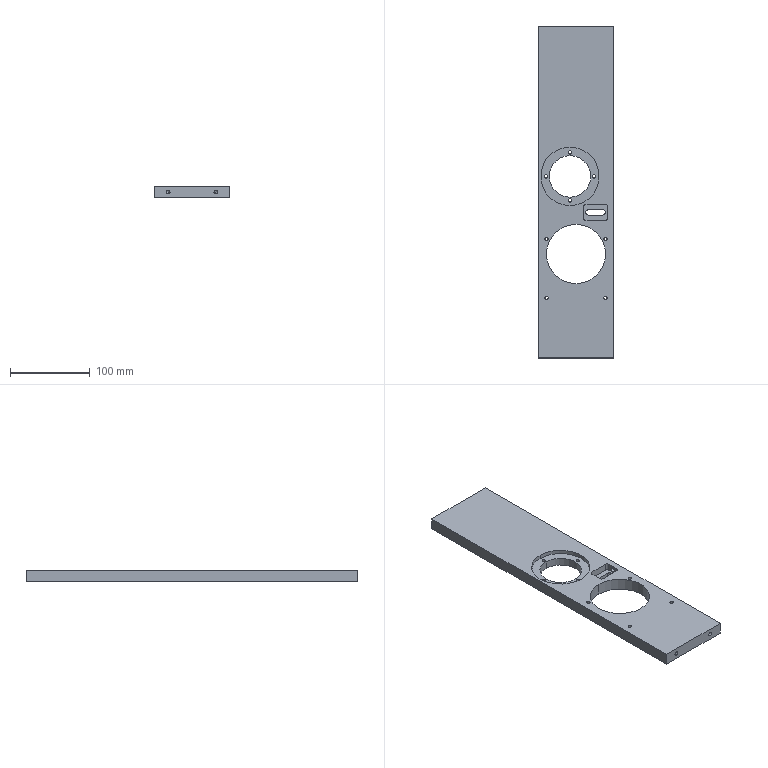Component | SolidWorks | 8TC-A15004-D0-02A-2 | 1 solid | 76 faces | box 95 x 415 x 15 mm | volume 474411 mm3 | cylinder 46 | cone 16 | plane 14 | commonest cylinder face diameters 5 x18 4.2 x16 6 x4 73 x2 74 x2 52 x2 6.5 x2 | material #45
build123d program:
from build123d import *

# Parameters (mm, degrees)
SKETCH1_W             = 95
SKETCH1_H             = 415
BOSS_EXTRUDE1_DEPTH   = 7.5
SKETCH3_R             = 26
CUT_EXTRUDE2_DEPTH    = 214.395
SKETCH4_R             = 37
CUT_EXTRUDE3_DEPTH    = 214.395
SKETCH5_R             = 36.5
CUT_EXTRUDE4_DEPTH    = 5
M6_TAPPED_HOLE1_D     = 5
M6_TAPPED_HOLE1_DEPTH = 15
M6_TAPPED_HOLE1_TIP   = 1.502
M6_TAPPED_HOLE2_D     = 5
M6_TAPPED_HOLE2_DEPTH = 15
M6_TAPPED_HOLE2_TIP   = 1.502
M5_TAPPED_HOLE1_D     = 4.2
CIRPATTERN1_COUNT     = 4
M6_TAPPED_HOLE5_D     = 5
M6_TAPPED_HOLE5_DEPTH = 15
M6_TAPPED_HOLE5_TIP   = 1.502
CUT_EXTRUDE5_DEPTH    = 9
CUT_EXTRUDE6_DEPTH    = 214.058
M6_TAPPED_HOLE4_D     = 5
M6_TAPPED_HOLE4_DEPTH = 8
M5_TAPPED_HOLE2_D     = 4.2
M6_TAPPED_HOLE6_D     = 5
M6_TAPPED_HOLE6_DEPTH = 17
M6_TAPPED_HOLE6_TIP   = 1.502


with BuildPart() as part:
    # Sketch1 → Boss-Extrude1 (new, symmetric)
    with BuildSketch(Plane(origin=(0, 0, 0), x_dir=(1, 0, 0), z_dir=(0, 1, 0))):
        Rectangle(SKETCH1_W, SKETCH1_H)
    extrude(amount=BOSS_EXTRUDE1_DEPTH, both=True)

    # Sketch3 → Cut-Extrude2 (cut, through all)
    with BuildSketch(Plane.XZ.offset(7.5)):
        with Locations(Location((7.5, -19.5, 0), (0, 0, 270))):
            Circle(SKETCH3_R)
    extrude(amount=-CUT_EXTRUDE2_DEPTH, mode=Mode.SUBTRACT)

    # Sketch4 → Cut-Extrude3 (cut, through all)
    with BuildSketch(Plane.XZ.offset(7.5)):
        with Locations(Location((0, 77.5, 0), (0, 0, 270))):
            Circle(SKETCH4_R)
    extrude(amount=-CUT_EXTRUDE3_DEPTH, mode=Mode.SUBTRACT)

    # Sketch5 → Cut-Extrude4 (cut)
    with BuildSketch(Plane.XZ.offset(7.5)):
        with Locations(Location((7.5, -19.5, 0), (0, 0, 270))):
            Circle(SKETCH5_R)
    extrude(amount=-CUT_EXTRUDE4_DEPTH, mode=Mode.SUBTRACT)

    # M6 Tapped Hole1
    with Locations(Plane.XY.offset(207.5)):
        with Locations((-30, 0), (30, 0)):
            Hole(M6_TAPPED_HOLE1_D / 2, depth=M6_TAPPED_HOLE1_DEPTH)
            with Locations((0, 0, -(M6_TAPPED_HOLE1_DEPTH + M6_TAPPED_HOLE1_TIP / 2))):  # 118° drill point
                Cone(0, M6_TAPPED_HOLE1_D / 2, M6_TAPPED_HOLE1_TIP, mode=Mode.SUBTRACT)

    # M6 Tapped Hole2
    with Locations(Plane(origin=(0, 0, -207.5), x_dir=(-1, 0, 0), z_dir=(0, 0, -1))):
        with Locations((-30, 0), (30, 0)):
            Hole(M6_TAPPED_HOLE2_D / 2, depth=M6_TAPPED_HOLE2_DEPTH)
            with Locations((0, 0, -(M6_TAPPED_HOLE2_DEPTH + M6_TAPPED_HOLE2_TIP / 2))):  # 118° drill point
                Cone(0, M6_TAPPED_HOLE2_D / 2, M6_TAPPED_HOLE2_TIP, mode=Mode.SUBTRACT)

    # M5 Tapped Hole1 (through all)
    with Locations(Plane(origin=(0, -2.5, 0), x_dir=(-1, 0, 0), z_dir=(0, -1, 0))):
        with Locations((-7.5, 49.5)):
            m5_tapped_hole1 = Hole(M5_TAPPED_HOLE1_D / 2)

    # CirPattern1: M5 Tapped Hole1 ×4 about axis
    cirpattern1_axis = Axis((7.5, 0, -19.5), (0, 1, 0))
    for i in range(1, CIRPATTERN1_COUNT):
        add(m5_tapped_hole1.rotate(cirpattern1_axis, i * 360 / CIRPATTERN1_COUNT), mode=Mode.SUBTRACT)

    # M6 Tapped Hole5
    with Locations(Plane.ZY.offset(47.5)):
        with Locations((-190.5, 0), (-140.5, 0)):
            Hole(M6_TAPPED_HOLE5_D / 2, depth=M6_TAPPED_HOLE5_DEPTH)
            with Locations((0, 0, -(M6_TAPPED_HOLE5_DEPTH + M6_TAPPED_HOLE5_TIP / 2))):  # 118° drill point
                Cone(0, M6_TAPPED_HOLE5_D / 2, M6_TAPPED_HOLE5_TIP, mode=Mode.SUBTRACT)

    # Sketch17 → Cut-Extrude5 (cut)
    with BuildSketch(Plane.XZ.offset(7.5)):
        with BuildLine():
            Line((-36.5, 15.5), (-12.5, 15.5))
            ThreePointArc((-12.5, 15.5), (-10.379, 16.379), (-9.5, 18.5))
            Line((-9.5, 18.5), (-9.5, 32.5))
            ThreePointArc((-9.5, 32.5), (-10.379, 34.621), (-12.5, 35.5))
            Line((-12.5, 35.5), (-36.5, 35.5))
            ThreePointArc((-36.5, 35.5), (-38.621, 34.621), (-39.5, 32.5))
            Line((-39.5, 32.5), (-39.5, 18.5))
            ThreePointArc((-39.5, 18.5), (-38.621, 16.379), (-36.5, 15.5))
        make_face()
    extrude(amount=-CUT_EXTRUDE5_DEPTH, mode=Mode.SUBTRACT)

    # Sketch18 → Cut-Extrude6 (cut, through all)
    with BuildSketch(Plane.XZ.offset(-1.5)):
        with BuildLine():
            Line((-33.5, 28.75), (-15.5, 28.75))
            ThreePointArc((-15.5, 28.75), (-12.25, 25.5), (-15.5, 22.25))
            Line((-15.5, 22.25), (-33.5, 22.25))
            ThreePointArc((-33.5, 22.25), (-36.75, 25.5), (-33.5, 28.75))
        make_face()
    extrude(amount=-CUT_EXTRUDE6_DEPTH, mode=Mode.SUBTRACT)

    # M6 Tapped Hole4
    with Locations(Plane.ZY.offset(47.5)):
        with Locations((25.5, -2.5)):
            Hole(M6_TAPPED_HOLE4_D / 2, depth=M6_TAPPED_HOLE4_DEPTH)

    # M5 Tapped Hole2 (through all)
    with Locations(Plane(origin=(0, -7.5, 0), x_dir=(-1, 0, 0), z_dir=(0, -1, 0))):
        with Locations((36.77, -132.27), (-36.77, -132.27), (-36.77, -58.73), (36.77, -58.73)):
            Hole(M5_TAPPED_HOLE2_D / 2)

    # M6 Tapped Hole6
    with Locations(Plane.ZY.offset(47.5)):
        with Locations((-125.5, 0), (-175.5, 0)):
            Hole(M6_TAPPED_HOLE6_D / 2, depth=M6_TAPPED_HOLE6_DEPTH)
            with Locations((0, 0, -(M6_TAPPED_HOLE6_DEPTH + M6_TAPPED_HOLE6_TIP / 2))):  # 118° drill point
                Cone(0, M6_TAPPED_HOLE6_D / 2, M6_TAPPED_HOLE6_TIP, mode=Mode.SUBTRACT)


solid = part.part

# Placed as in the assembly
solid = solid.moved(Location((0, 215, 117.5), (90, 0, -180)))